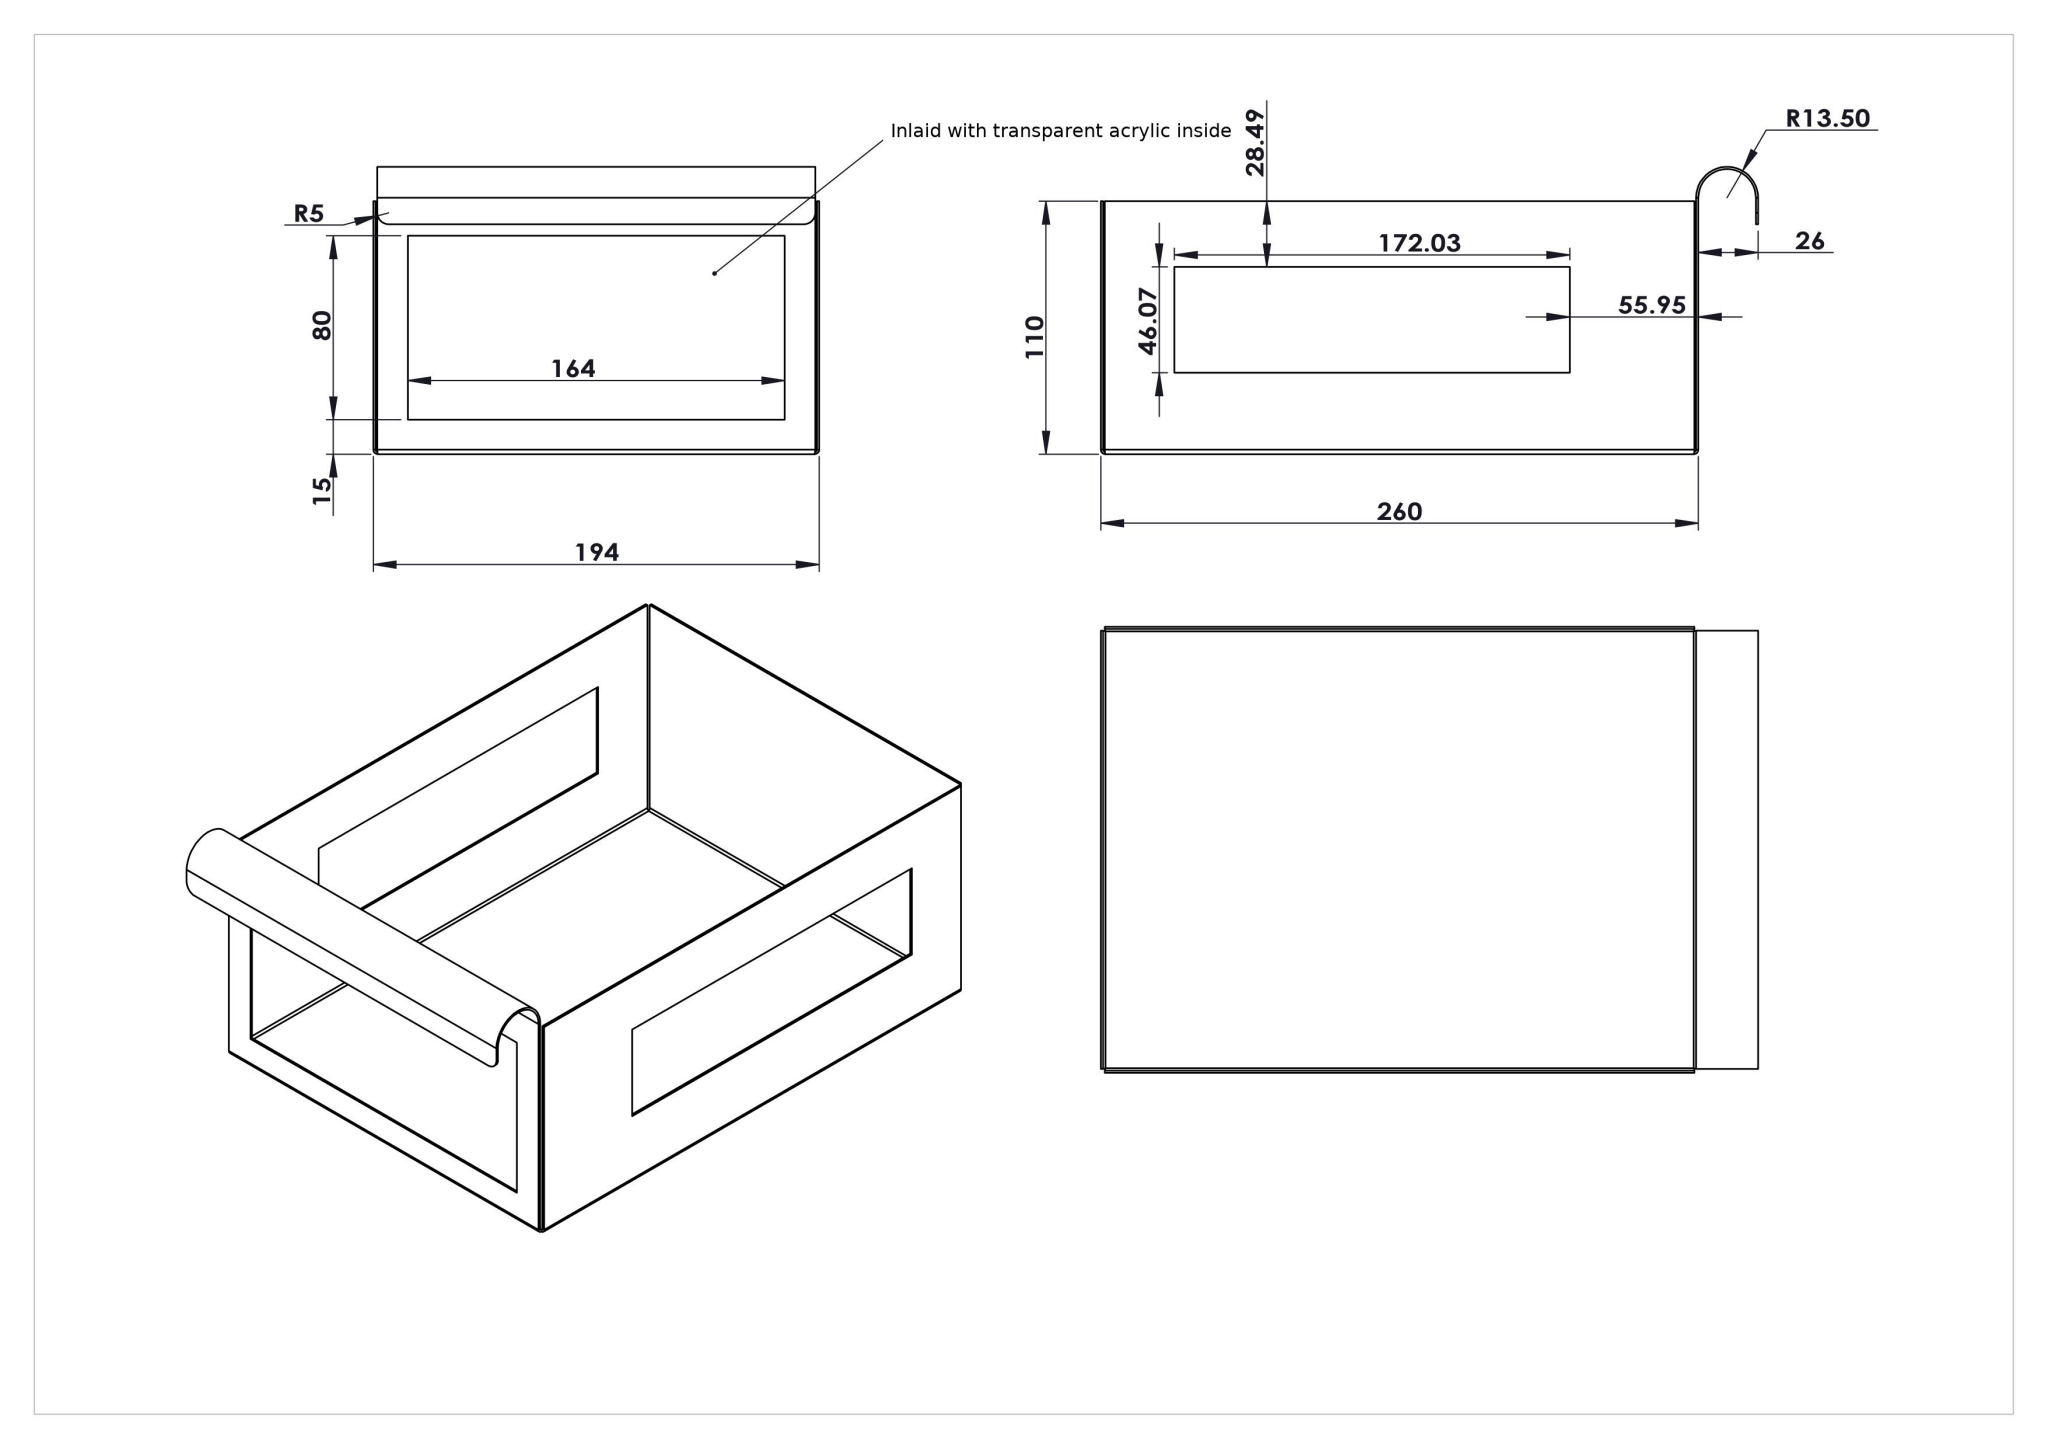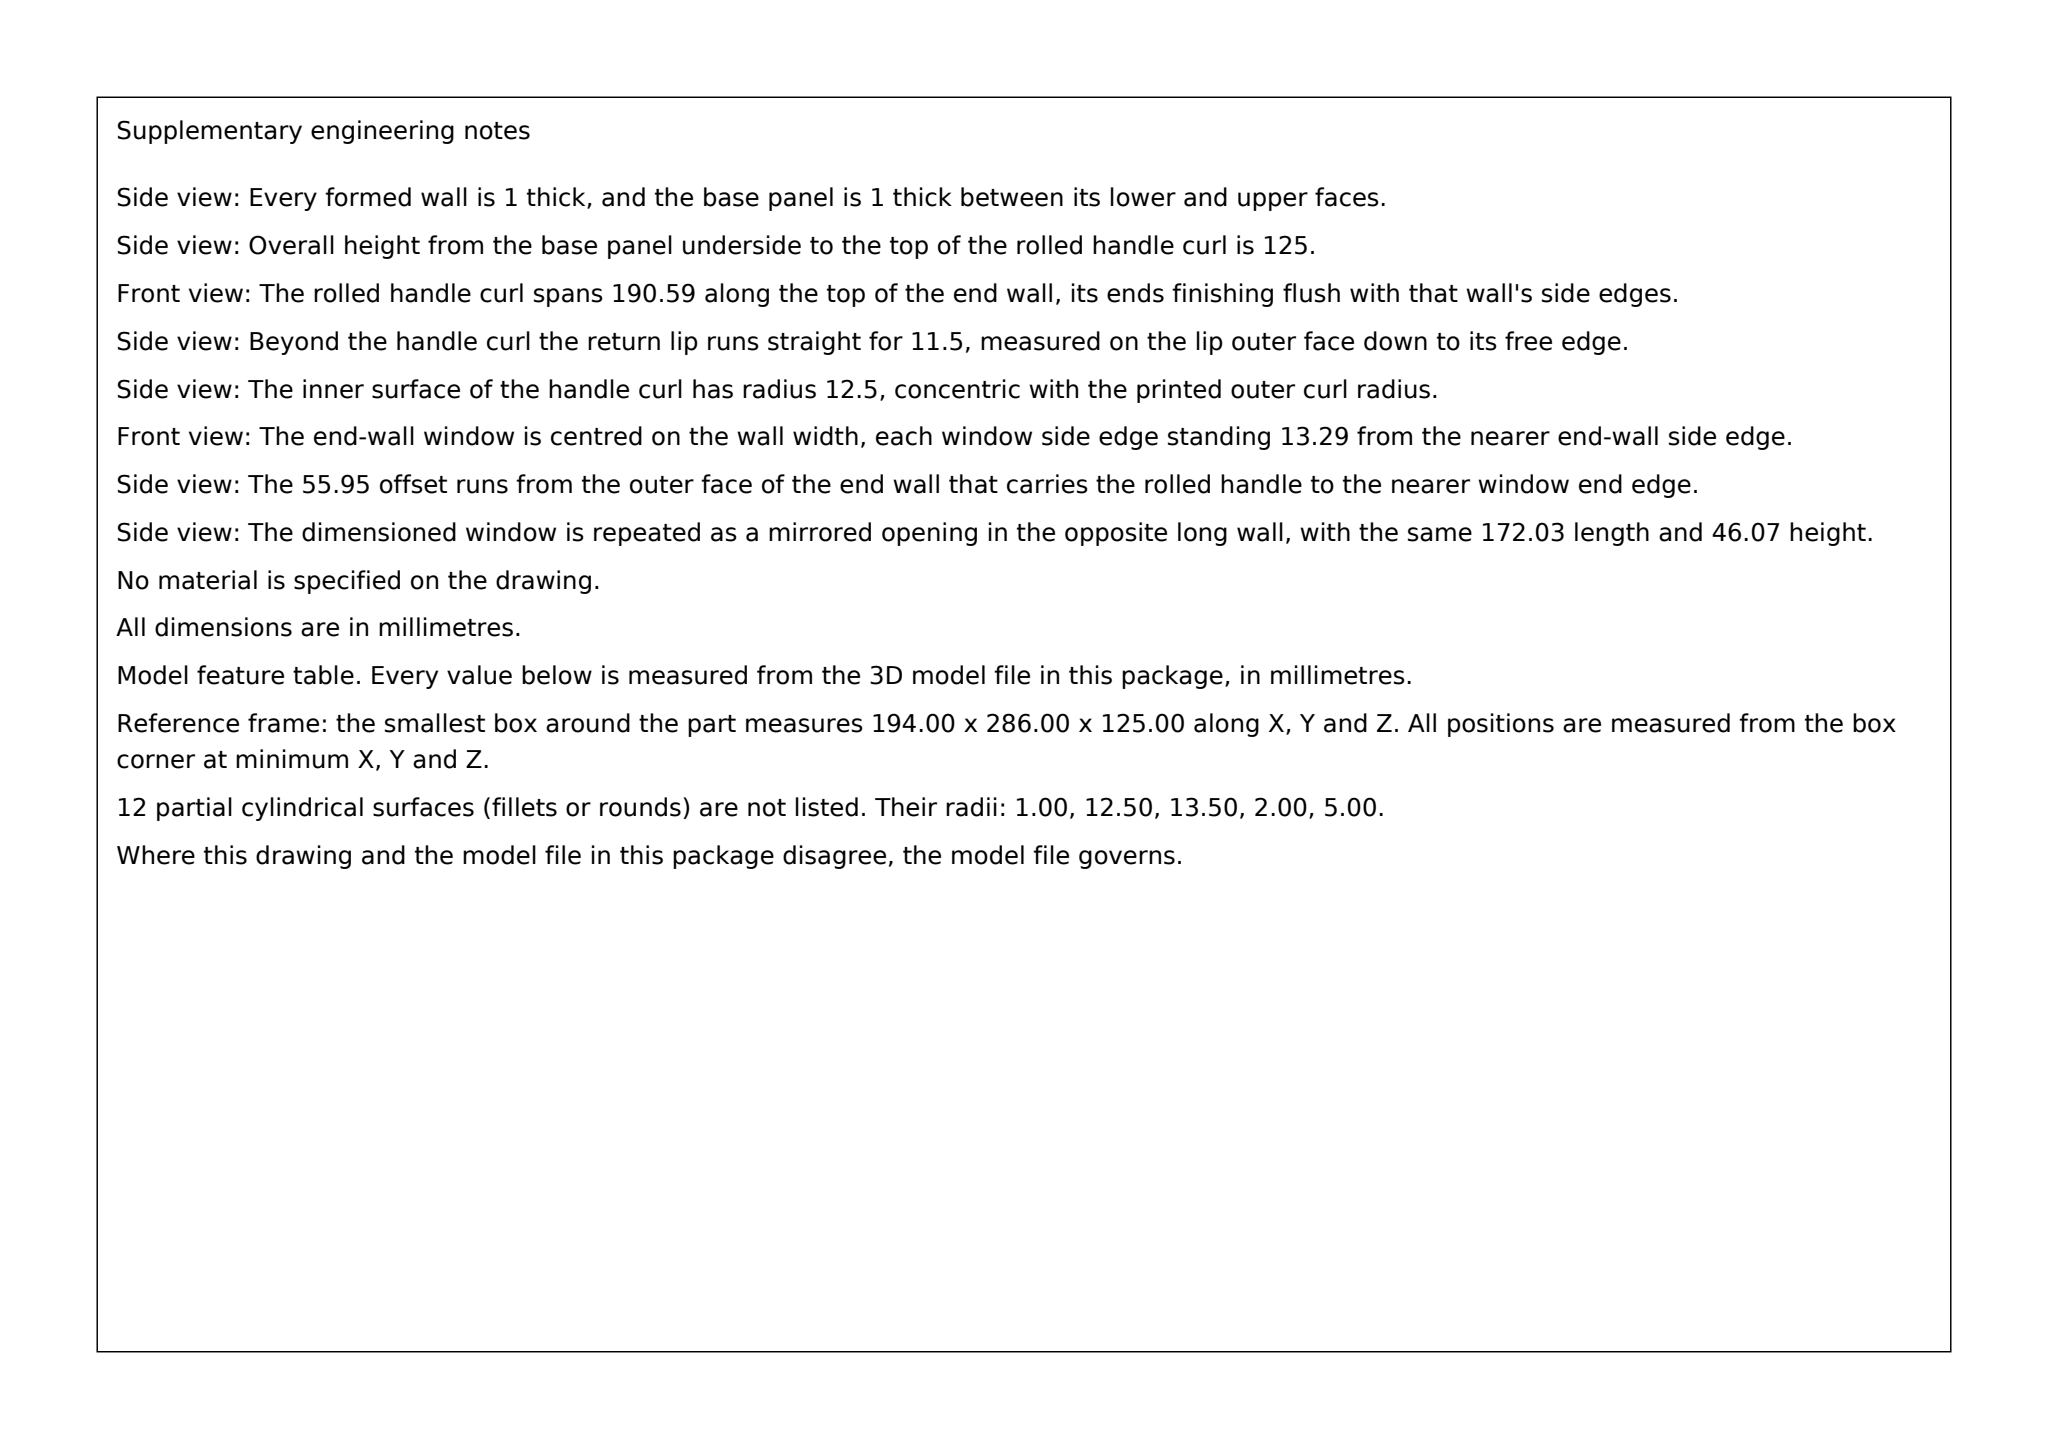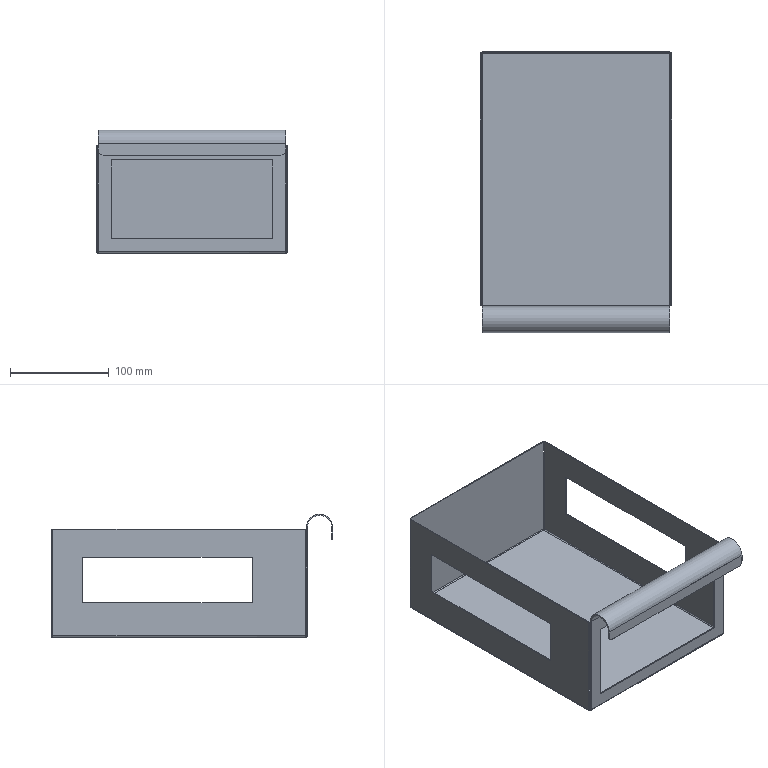Part | SolidWorks | mm | 1 solid | 60 faces | box 194 x 286 x 125 mm | volume 128614 mm3 | plane 40 | cylinder 12 | spline 8 | commonest cylinder face diameters 4 x4 2 x4 10 x2 27 x1 25 x1
Drawing notes:
UNSPECIFIED BEND RADII: R1 INSIDE, R2 OUTSIDE (4X BOTTOM BENDS) | from the solid: Cyl dia 2 (inner) & dia 4 (outer) at y=28/284 and x=2.01/192.01, all at z=2.01
ACRYLIC INLAY 0.71 THK ON INNER FACE OF ALL 4 WALLS | from the solid: Panels: x planes 1.01->1.72 & 193.01->192.30; y planes 27.00->27.71 & 285.00->284.29
HOOK RETURN LEG ENDS 25 BELOW 125 TOP = 10 BELOW 110 WALL TOP | from the solid: z=100.01 free end plane; overall z=125.01; wall top z=110.01
2X SIDE WALL CUT-OUT 172.03 X 46.07, SYM BOTH SIDES | from the solid: Identical openings at x=1.72/192.30 walls, z=35.45 to 81.52
FRONT CUT-OUT 164 WIDE SYM ABT CL: 15 FROM EA SIDE EDGE | from the solid: x-planes 15.01 and 179.01 bound 164 cut-out in 194.02 overall width; 194.02-179.01=15.01
HOOK BAR R13.50 FORM, 190.59 LG, SYM ABT PART CL: ENDS 1.72 FROM EACH OUTER SIDE FACE (X 1.72 TO X 192.30) | from the solid: cylinders dia 27/25 axis x, pos y13.5 z111.51, length 190.59; axis_planes x=1.72 (4) and x=192.30 (4); bbox_x 194.02
HOOK RETURN LEG 1 THK: OUTER FACE AT Y=0, INNER FACE Y=1, 25 CLEAR TO WALL OUTER FACE (Y=26); LEG END AT Z=100.01 (25 BELOW 125 TOP) | from the solid: axis_planes y=0.0, y=1.0, y=26.0, y=27.0; z=100.01; z=110.01; bbox_z 125.01
BALLOON 4 = HOOK BAR LENGTH 190.59; BALLOON 1 = 1 THK WALL; BALLOON 2 = 125 OVERALL HEIGHT | from the solid: cylinder dia 27 axis x length 190.59; axis_planes x=0.01/1.01 and x=193.01/194.01 (1 thk); bbox_xyz z = 125.01